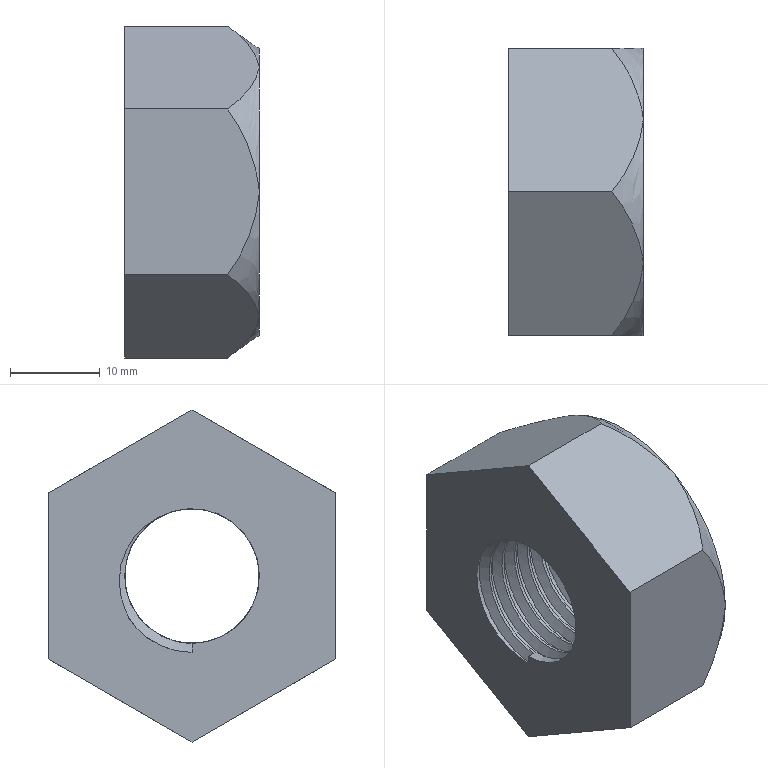Component | NX | NUT_7 | 1 solid | 20 faces | volume 10130 mm3 | plane 10 | other 6 | cylinder 2 | spline 2 | commonest cylinder face diameters 15 x1 17 x1